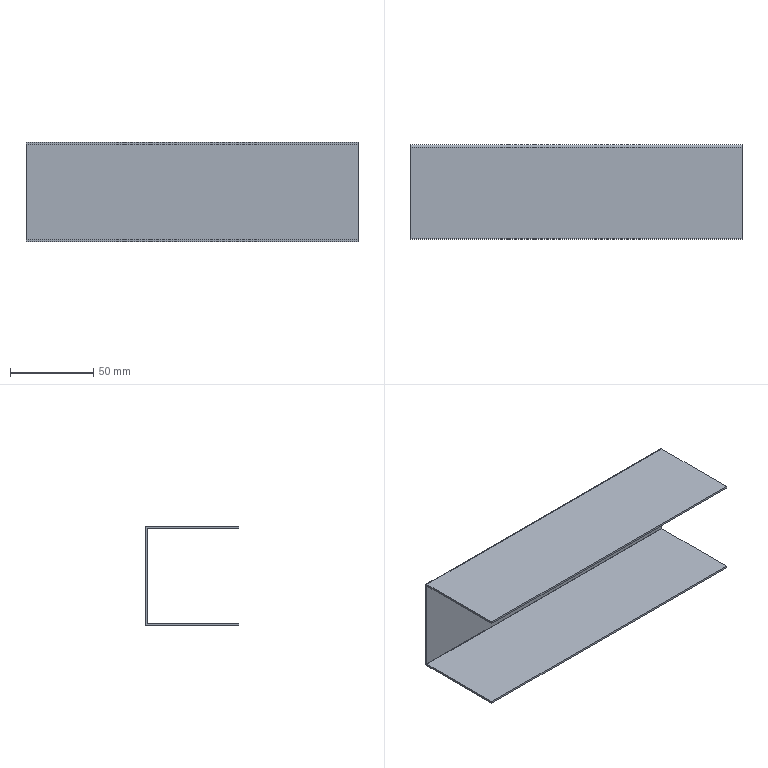Component | SolidWorks | WeldmentDrawing-1_DrawerBoxBracket-1 | 1 solid | 22 faces | box 200 x 56.6 x 60 mm | volume 40848 mm3 | plane 18 | cylinder 4 | commonest cylinder face diameters 2.6 x2 0.2 x2
STEP:
#1=CARTESIAN_POINT('',(-5.191,-11.825,-0.3425));
#2=VERTEX_POINT('',#1);
#3=CARTESIAN_POINT('',(-5.191,-11.825,1.917));
#4=VERTEX_POINT('',#3);
#5=CARTESIAN_POINT('',(-5.191,-11.825,1.969));
#6=DIRECTION('',(0.,0.,1.));
#7=VECTOR('',#6,39.37);
#8=LINE('',#5,#7);
#9=EDGE_CURVE('',#2,#4,#8,.T.);
#10=ORIENTED_EDGE('',*,*,#9,.F.);
#11=CARTESIAN_POINT('',(2.683,-11.825,-0.3425));
#12=VERTEX_POINT('',#11);
#13=CARTESIAN_POINT('',(2.683,-11.825,-0.3425));
#14=DIRECTION('',(-1.,0.,0.));
#15=VECTOR('',#14,39.37);
#16=LINE('',#13,#15);
#17=EDGE_CURVE('',#12,#2,#16,.T.);
#18=ORIENTED_EDGE('',*,*,#17,.F.);
#19=CARTESIAN_POINT('',(2.683,-11.825,1.917));
#20=VERTEX_POINT('',#19);
#21=CARTESIAN_POINT('',(2.683,-11.825,1.969));
#22=DIRECTION('',(0.,0.,-1.));
#23=VECTOR('',#22,39.37);
#24=LINE('',#21,#23);
#25=EDGE_CURVE('',#20,#12,#24,.T.);
#26=ORIENTED_EDGE('',*,*,#25,.F.);
#27=CARTESIAN_POINT('',(-5.191,-11.825,1.917));
#28=DIRECTION('',(1.,0.,0.));
#29=VECTOR('',#28,39.37);
#30=LINE('',#27,#29);
#31=EDGE_CURVE('',#4,#20,#30,.T.);
#32=ORIENTED_EDGE('',*,*,#31,.F.);
#33=EDGE_LOOP('',(#10,#18,#26,#32));
#34=FACE_OUTER_BOUND('',#33,.T.);
#35=CARTESIAN_POINT('',(-2.423,-11.825,0.8285));
#36=DIRECTION('',(0.,-1.,0.));
#37=DIRECTION('',(0.,0.,-1.));
#38=AXIS2_PLACEMENT_3D('',#35,#36,#37);
#39=PLANE('',#38);
#40=ADVANCED_FACE('',(#34),#39,.T.);
#41=CARTESIAN_POINT('',(2.683,-11.778,-0.3425));
#42=VERTEX_POINT('',#41);
#43=CARTESIAN_POINT('',(-5.191,-11.778,-0.3425));
#44=VERTEX_POINT('',#43);
#45=CARTESIAN_POINT('',(2.683,-11.778,-0.3425));
#46=DIRECTION('',(-1.,0.,0.));
#47=VECTOR('',#46,39.37);
#48=LINE('',#45,#47);
#49=EDGE_CURVE('',#42,#44,#48,.T.);
#50=ORIENTED_EDGE('',*,*,#49,.T.);
#51=CARTESIAN_POINT('',(-5.191,-11.778,1.917));
#52=VERTEX_POINT('',#51);
#53=CARTESIAN_POINT('',(-5.191,-11.778,1.969));
#54=DIRECTION('',(0.,0.,1.));
#55=VECTOR('',#54,39.37);
#56=LINE('',#53,#55);
#57=EDGE_CURVE('',#44,#52,#56,.T.);
#58=ORIENTED_EDGE('',*,*,#57,.T.);
#59=CARTESIAN_POINT('',(2.683,-11.778,1.917));
#60=VERTEX_POINT('',#59);
#61=CARTESIAN_POINT('',(-5.191,-11.778,1.917));
#62=DIRECTION('',(1.,0.,0.));
#63=VECTOR('',#62,39.37);
#64=LINE('',#61,#63);
#65=EDGE_CURVE('',#52,#60,#64,.T.);
#66=ORIENTED_EDGE('',*,*,#65,.T.);
#67=CARTESIAN_POINT('',(2.683,-11.778,1.969));
#68=DIRECTION('',(0.,0.,-1.));
#69=VECTOR('',#68,39.37);
#70=LINE('',#67,#69);
#71=EDGE_CURVE('',#60,#42,#70,.T.);
#72=ORIENTED_EDGE('',*,*,#71,.T.);
#73=EDGE_LOOP('',(#50,#58,#66,#72));
#74=FACE_OUTER_BOUND('',#73,.T.);
#75=CARTESIAN_POINT('',(-2.423,-11.778,0.8285));
#76=DIRECTION('',(0.,-1.,0.));
#77=DIRECTION('',(0.,0.,-1.));
#78=AXIS2_PLACEMENT_3D('',#75,#76,#77);
#79=PLANE('',#78);
#80=ADVANCED_FACE('',(#74),#79,.F.);
#81=ORIENTED_EDGE('',*,*,#25,.T.);
#82=CARTESIAN_POINT('',(2.683,-11.825,-0.3425));
#83=DIRECTION('',(0.,1.,0.));
#84=VECTOR('',#83,39.37);
#85=LINE('',#82,#84);
#86=EDGE_CURVE('',#12,#42,#85,.T.);
#87=ORIENTED_EDGE('',*,*,#86,.T.);
#88=ORIENTED_EDGE('',*,*,#71,.F.);
#89=CARTESIAN_POINT('',(2.683,-11.825,1.917));
#90=DIRECTION('',(0.,1.,0.));
#91=VECTOR('',#90,39.37);
#92=LINE('',#89,#91);
#93=EDGE_CURVE('',#20,#60,#92,.T.);
#94=ORIENTED_EDGE('',*,*,#93,.F.);
#95=EDGE_LOOP('',(#81,#87,#88,#94));
#96=FACE_OUTER_BOUND('',#95,.T.);
#97=CARTESIAN_POINT('',(2.683,-11.825,1.969));
#98=DIRECTION('',(1.,0.,0.));
#99=DIRECTION('',(0.,0.,-1.));
#100=AXIS2_PLACEMENT_3D('',#97,#98,#99);
#101=PLANE('',#100);
#102=ADVANCED_FACE('',(#96),#101,.T.);
#103=CARTESIAN_POINT('',(-5.191,-11.825,-0.3425));
#104=DIRECTION('',(0.,1.,0.));
#105=VECTOR('',#104,39.37);
#106=LINE('',#103,#105);
#107=EDGE_CURVE('',#2,#44,#106,.T.);
#108=ORIENTED_EDGE('',*,*,#107,.F.);
#109=ORIENTED_EDGE('',*,*,#9,.T.);
#110=CARTESIAN_POINT('',(-5.191,-11.825,1.917));
#111=DIRECTION('',(0.,1.,0.));
#112=VECTOR('',#111,39.37);
#113=LINE('',#110,#112);
#114=EDGE_CURVE('',#4,#52,#113,.T.);
#115=ORIENTED_EDGE('',*,*,#114,.T.);
#116=ORIENTED_EDGE('',*,*,#57,.F.);
#117=EDGE_LOOP('',(#108,#109,#115,#116));
#118=FACE_OUTER_BOUND('',#117,.T.);
#119=CARTESIAN_POINT('',(-5.191,-11.825,1.969));
#120=DIRECTION('',(-1.,0.,0.));
#121=DIRECTION('',(0.,0.,1.));
#122=AXIS2_PLACEMENT_3D('',#119,#120,#121);
#123=PLANE('',#122);
#124=ADVANCED_FACE('',(#118),#123,.T.);
#125=CARTESIAN_POINT('',(2.683,-11.829,1.921));
#126=VERTEX_POINT('',#125);
#127=CARTESIAN_POINT('',(2.683,-11.829,1.969));
#128=VERTEX_POINT('',#127);
#129=CARTESIAN_POINT('',(2.683,-11.829,1.969));
#130=DIRECTION('',(0.,0.,1.));
#131=VECTOR('',#130,39.37);
#132=LINE('',#129,#131);
#133=EDGE_CURVE('',#126,#128,#132,.T.);
#134=ORIENTED_EDGE('',*,*,#133,.F.);
#135=CARTESIAN_POINT('',(2.683,-11.829,1.917));
#136=DIRECTION('',(1.,0.,0.));
#137=DIRECTION('',(0.,0.,1.));
#138=AXIS2_PLACEMENT_3D('',#135,#136,#137);
#139=CIRCLE('',#138,0.003937);
#140=EDGE_CURVE('',#20,#126,#139,.T.);
#141=ORIENTED_EDGE('',*,*,#140,.F.);
#142=ORIENTED_EDGE('',*,*,#93,.T.);
#143=CARTESIAN_POINT('',(2.683,-11.829,1.917));
#144=DIRECTION('',(1.,0.,0.));
#145=DIRECTION('',(0.,-0.,1.));
#146=AXIS2_PLACEMENT_3D('',#143,#144,#145);
#147=CIRCLE('',#146,0.05118);
#148=EDGE_CURVE('',#60,#128,#147,.T.);
#149=ORIENTED_EDGE('',*,*,#148,.T.);
#150=EDGE_LOOP('',(#134,#141,#142,#149));
#151=FACE_OUTER_BOUND('',#150,.T.);
#152=CARTESIAN_POINT('',(2.683,-11.829,1.917));
#153=DIRECTION('',(1.,0.,0.));
#154=DIRECTION('',(0.,0.,-1.));
#155=AXIS2_PLACEMENT_3D('',#152,#153,#154);
#156=PLANE('',#155);
#157=ADVANCED_FACE('',(#151),#156,.T.);
#158=CARTESIAN_POINT('',(-5.191,-11.829,1.921));
#159=VERTEX_POINT('',#158);
#160=CARTESIAN_POINT('',(-5.191,-11.829,1.917));
#161=DIRECTION('',(-1.,0.,0.));
#162=DIRECTION('',(0.,0.,1.));
#163=AXIS2_PLACEMENT_3D('',#160,#161,#162);
#164=CIRCLE('',#163,0.003937);
#165=EDGE_CURVE('',#159,#4,#164,.T.);
#166=ORIENTED_EDGE('',*,*,#165,.F.);
#167=CARTESIAN_POINT('',(-5.191,-11.829,1.969));
#168=VERTEX_POINT('',#167);
#169=CARTESIAN_POINT('',(-5.191,-11.829,1.921));
#170=DIRECTION('',(0.,0.,1.));
#171=VECTOR('',#170,39.37);
#172=LINE('',#169,#171);
#173=EDGE_CURVE('',#159,#168,#172,.T.);
#174=ORIENTED_EDGE('',*,*,#173,.T.);
#175=CARTESIAN_POINT('',(-5.191,-11.829,1.917));
#176=DIRECTION('',(-1.,0.,0.));
#177=DIRECTION('',(0.,0.,1.));
#178=AXIS2_PLACEMENT_3D('',#175,#176,#177);
#179=CIRCLE('',#178,0.05118);
#180=EDGE_CURVE('',#168,#52,#179,.T.);
#181=ORIENTED_EDGE('',*,*,#180,.T.);
#182=ORIENTED_EDGE('',*,*,#114,.F.);
#183=EDGE_LOOP('',(#166,#174,#181,#182));
#184=FACE_OUTER_BOUND('',#183,.T.);
#185=CARTESIAN_POINT('',(-5.191,-11.829,1.917));
#186=DIRECTION('',(1.,0.,0.));
#187=DIRECTION('',(0.,0.,-1.));
#188=AXIS2_PLACEMENT_3D('',#185,#186,#187);
#189=PLANE('',#188);
#190=ADVANCED_FACE('',(#184),#189,.F.);
#191=ORIENTED_EDGE('',*,*,#65,.F.);
#192=ORIENTED_EDGE('',*,*,#180,.F.);
#193=CARTESIAN_POINT('',(-2.423,-11.829,1.969));
#194=DIRECTION('',(-1.,0.,0.));
#195=VECTOR('',#194,39.37);
#196=LINE('',#193,#195);
#197=EDGE_CURVE('',#128,#168,#196,.T.);
#198=ORIENTED_EDGE('',*,*,#197,.F.);
#199=ORIENTED_EDGE('',*,*,#148,.F.);
#200=EDGE_LOOP('',(#191,#192,#198,#199));
#201=FACE_OUTER_BOUND('',#200,.T.);
#202=CARTESIAN_POINT('',(-5.191,-11.829,1.917));
#203=DIRECTION('',(-1.,0.,0.));
#204=DIRECTION('',(0.,0.,1.));
#205=AXIS2_PLACEMENT_3D('',#202,#203,#204);
#206=CYLINDRICAL_SURFACE('',#205,0.05118);
#207=ADVANCED_FACE('',(#201),#206,.T.);
#208=ORIENTED_EDGE('',*,*,#31,.T.);
#209=ORIENTED_EDGE('',*,*,#140,.T.);
#210=CARTESIAN_POINT('',(2.683,-11.829,1.921));
#211=DIRECTION('',(-1.,0.,0.));
#212=VECTOR('',#211,39.37);
#213=LINE('',#210,#212);
#214=EDGE_CURVE('',#126,#159,#213,.T.);
#215=ORIENTED_EDGE('',*,*,#214,.T.);
#216=ORIENTED_EDGE('',*,*,#165,.T.);
#217=EDGE_LOOP('',(#208,#209,#215,#216));
#218=FACE_OUTER_BOUND('',#217,.T.);
#219=CARTESIAN_POINT('',(-5.191,-11.829,1.917));
#220=DIRECTION('',(-1.,0.,0.));
#221=DIRECTION('',(0.,0.,1.));
#222=AXIS2_PLACEMENT_3D('',#219,#220,#221);
#223=CYLINDRICAL_SURFACE('',#222,0.003937);
#224=ADVANCED_FACE('',(#218),#223,.F.);
#225=CARTESIAN_POINT('',(-5.191,-14.006,1.969));
#226=VERTEX_POINT('',#225);
#227=CARTESIAN_POINT('',(-5.191,-11.825,1.969));
#228=DIRECTION('',(0.,1.,-0.));
#229=VECTOR('',#228,39.37);
#230=LINE('',#227,#229);
#231=EDGE_CURVE('',#226,#168,#230,.T.);
#232=ORIENTED_EDGE('',*,*,#231,.T.);
#233=ORIENTED_EDGE('',*,*,#173,.F.);
#234=CARTESIAN_POINT('',(-5.191,-14.006,1.921));
#235=VERTEX_POINT('',#234);
#236=CARTESIAN_POINT('',(-5.191,-11.778,1.921));
#237=DIRECTION('',(0.,1.,-0.));
#238=VECTOR('',#237,39.37);
#239=LINE('',#236,#238);
#240=EDGE_CURVE('',#235,#159,#239,.T.);
#241=ORIENTED_EDGE('',*,*,#240,.F.);
#242=CARTESIAN_POINT('',(-5.191,-14.006,1.969));
#243=DIRECTION('',(0.,-0.,-1.));
#244=VECTOR('',#243,39.37);
#245=LINE('',#242,#244);
#246=EDGE_CURVE('',#226,#235,#245,.T.);
#247=ORIENTED_EDGE('',*,*,#246,.F.);
#248=EDGE_LOOP('',(#232,#233,#241,#247));
#249=FACE_OUTER_BOUND('',#248,.T.);
#250=CARTESIAN_POINT('',(-5.191,-11.825,1.969));
#251=DIRECTION('',(-1.,0.,0.));
#252=DIRECTION('',(0.,0.,1.));
#253=AXIS2_PLACEMENT_3D('',#250,#251,#252);
#254=PLANE('',#253);
#255=ADVANCED_FACE('',(#249),#254,.T.);
#256=CARTESIAN_POINT('',(2.683,-14.006,1.921));
#257=VERTEX_POINT('',#256);
#258=CARTESIAN_POINT('',(2.683,-11.778,1.921));
#259=DIRECTION('',(0.,-1.,0.));
#260=VECTOR('',#259,39.37);
#261=LINE('',#258,#260);
#262=EDGE_CURVE('',#126,#257,#261,.T.);
#263=ORIENTED_EDGE('',*,*,#262,.F.);
#264=ORIENTED_EDGE('',*,*,#133,.T.);
#265=CARTESIAN_POINT('',(2.683,-14.006,1.969));
#266=VERTEX_POINT('',#265);
#267=CARTESIAN_POINT('',(2.683,-14.006,1.969));
#268=DIRECTION('',(0.,-1.,0.));
#269=VECTOR('',#268,39.37);
#270=LINE('',#267,#269);
#271=EDGE_CURVE('',#128,#266,#270,.T.);
#272=ORIENTED_EDGE('',*,*,#271,.T.);
#273=CARTESIAN_POINT('',(2.683,-14.006,1.969));
#274=DIRECTION('',(0.,-0.,-1.));
#275=VECTOR('',#274,39.37);
#276=LINE('',#273,#275);
#277=EDGE_CURVE('',#266,#257,#276,.T.);
#278=ORIENTED_EDGE('',*,*,#277,.T.);
#279=EDGE_LOOP('',(#263,#264,#272,#278));
#280=FACE_OUTER_BOUND('',#279,.T.);
#281=CARTESIAN_POINT('',(2.683,-14.006,1.969));
#282=DIRECTION('',(1.,0.,0.));
#283=DIRECTION('',(0.,0.,-1.));
#284=AXIS2_PLACEMENT_3D('',#281,#282,#283);
#285=PLANE('',#284);
#286=ADVANCED_FACE('',(#280),#285,.T.);
#287=ORIENTED_EDGE('',*,*,#271,.F.);
#288=ORIENTED_EDGE('',*,*,#197,.T.);
#289=ORIENTED_EDGE('',*,*,#231,.F.);
#290=CARTESIAN_POINT('',(-5.191,-14.006,1.969));
#291=DIRECTION('',(-1.,0.,0.));
#292=VECTOR('',#291,39.37);
#293=LINE('',#290,#292);
#294=EDGE_CURVE('',#266,#226,#293,.T.);
#295=ORIENTED_EDGE('',*,*,#294,.F.);
#296=EDGE_LOOP('',(#287,#288,#289,#295));
#297=FACE_OUTER_BOUND('',#296,.T.);
#298=CARTESIAN_POINT('',(-2.423,-11.778,1.969));
#299=DIRECTION('',(0.,0.,1.));
#300=DIRECTION('',(0.,-1.,0.));
#301=AXIS2_PLACEMENT_3D('',#298,#299,#300);
#302=PLANE('',#301);
#303=ADVANCED_FACE('',(#297),#302,.T.);
#304=ORIENTED_EDGE('',*,*,#214,.F.);
#305=ORIENTED_EDGE('',*,*,#262,.T.);
#306=CARTESIAN_POINT('',(-2.423,-14.006,1.921));
#307=DIRECTION('',(-1.,0.,0.));
#308=VECTOR('',#307,39.37);
#309=LINE('',#306,#308);
#310=EDGE_CURVE('',#257,#235,#309,.T.);
#311=ORIENTED_EDGE('',*,*,#310,.T.);
#312=ORIENTED_EDGE('',*,*,#240,.T.);
#313=EDGE_LOOP('',(#304,#305,#311,#312));
#314=FACE_OUTER_BOUND('',#313,.T.);
#315=CARTESIAN_POINT('',(-2.423,-11.778,1.921));
#316=DIRECTION('',(0.,0.,1.));
#317=DIRECTION('',(0.,-1.,0.));
#318=AXIS2_PLACEMENT_3D('',#315,#316,#317);
#319=PLANE('',#318);
#320=ADVANCED_FACE('',(#314),#319,.F.);
#321=ORIENTED_EDGE('',*,*,#310,.F.);
#322=ORIENTED_EDGE('',*,*,#277,.F.);
#323=ORIENTED_EDGE('',*,*,#294,.T.);
#324=ORIENTED_EDGE('',*,*,#246,.T.);
#325=EDGE_LOOP('',(#321,#322,#323,#324));
#326=FACE_OUTER_BOUND('',#325,.T.);
#327=CARTESIAN_POINT('',(-5.191,-14.006,1.969));
#328=DIRECTION('',(0.,-1.,0.));
#329=DIRECTION('',(0.,-0.,-1.));
#330=AXIS2_PLACEMENT_3D('',#327,#328,#329);
#331=PLANE('',#330);
#332=ADVANCED_FACE('',(#326),#331,.T.);
#333=CARTESIAN_POINT('',(-5.191,-11.829,-0.3464));
#334=VERTEX_POINT('',#333);
#335=CARTESIAN_POINT('',(-5.191,-11.829,-0.3937));
#336=VERTEX_POINT('',#335);
#337=CARTESIAN_POINT('',(-5.191,-11.829,-0.3937));
#338=DIRECTION('',(0.,0.,-1.));
#339=VECTOR('',#338,39.37);
#340=LINE('',#337,#339);
#341=EDGE_CURVE('',#334,#336,#340,.T.);
#342=ORIENTED_EDGE('',*,*,#341,.F.);
#343=CARTESIAN_POINT('',(-5.191,-11.829,-0.3425));
#344=DIRECTION('',(-1.,0.,0.));
#345=DIRECTION('',(0.,0.,-1.));
#346=AXIS2_PLACEMENT_3D('',#343,#344,#345);
#347=CIRCLE('',#346,0.003937);
#348=EDGE_CURVE('',#2,#334,#347,.T.);
#349=ORIENTED_EDGE('',*,*,#348,.F.);
#350=ORIENTED_EDGE('',*,*,#107,.T.);
#351=CARTESIAN_POINT('',(-5.191,-11.829,-0.3425));
#352=DIRECTION('',(-1.,0.,0.));
#353=DIRECTION('',(0.,0.,-1.));
#354=AXIS2_PLACEMENT_3D('',#351,#352,#353);
#355=CIRCLE('',#354,0.05118);
#356=EDGE_CURVE('',#44,#336,#355,.T.);
#357=ORIENTED_EDGE('',*,*,#356,.T.);
#358=EDGE_LOOP('',(#342,#349,#350,#357));
#359=FACE_OUTER_BOUND('',#358,.T.);
#360=CARTESIAN_POINT('',(-5.191,-11.829,-0.3425));
#361=DIRECTION('',(-1.,0.,0.));
#362=DIRECTION('',(0.,0.,1.));
#363=AXIS2_PLACEMENT_3D('',#360,#361,#362);
#364=PLANE('',#363);
#365=ADVANCED_FACE('',(#359),#364,.T.);
#366=CARTESIAN_POINT('',(2.683,-11.829,-0.3464));
#367=VERTEX_POINT('',#366);
#368=CARTESIAN_POINT('',(2.683,-11.829,-0.3425));
#369=DIRECTION('',(1.,0.,0.));
#370=DIRECTION('',(0.,0.,-1.));
#371=AXIS2_PLACEMENT_3D('',#368,#369,#370);
#372=CIRCLE('',#371,0.003937);
#373=EDGE_CURVE('',#367,#12,#372,.T.);
#374=ORIENTED_EDGE('',*,*,#373,.F.);
#375=CARTESIAN_POINT('',(2.683,-11.829,-0.3937));
#376=VERTEX_POINT('',#375);
#377=CARTESIAN_POINT('',(2.683,-11.829,-0.3464));
#378=DIRECTION('',(0.,0.,-1.));
#379=VECTOR('',#378,39.37);
#380=LINE('',#377,#379);
#381=EDGE_CURVE('',#367,#376,#380,.T.);
#382=ORIENTED_EDGE('',*,*,#381,.T.);
#383=CARTESIAN_POINT('',(2.683,-11.829,-0.3425));
#384=DIRECTION('',(1.,0.,0.));
#385=DIRECTION('',(0.,0.,-1.));
#386=AXIS2_PLACEMENT_3D('',#383,#384,#385);
#387=CIRCLE('',#386,0.05118);
#388=EDGE_CURVE('',#376,#42,#387,.T.);
#389=ORIENTED_EDGE('',*,*,#388,.T.);
#390=ORIENTED_EDGE('',*,*,#86,.F.);
#391=EDGE_LOOP('',(#374,#382,#389,#390));
#392=FACE_OUTER_BOUND('',#391,.T.);
#393=CARTESIAN_POINT('',(2.683,-11.829,-0.3425));
#394=DIRECTION('',(-1.,0.,0.));
#395=DIRECTION('',(0.,0.,1.));
#396=AXIS2_PLACEMENT_3D('',#393,#394,#395);
#397=PLANE('',#396);
#398=ADVANCED_FACE('',(#392),#397,.F.);
#399=ORIENTED_EDGE('',*,*,#49,.F.);
#400=ORIENTED_EDGE('',*,*,#388,.F.);
#401=CARTESIAN_POINT('',(-5.191,-11.829,-0.3937));
#402=DIRECTION('',(-1.,0.,0.));
#403=VECTOR('',#402,39.37);
#404=LINE('',#401,#403);
#405=EDGE_CURVE('',#376,#336,#404,.T.);
#406=ORIENTED_EDGE('',*,*,#405,.T.);
#407=ORIENTED_EDGE('',*,*,#356,.F.);
#408=EDGE_LOOP('',(#399,#400,#406,#407));
#409=FACE_OUTER_BOUND('',#408,.T.);
#410=CARTESIAN_POINT('',(2.683,-11.829,-0.3425));
#411=DIRECTION('',(1.,0.,0.));
#412=DIRECTION('',(0.,0.,-1.));
#413=AXIS2_PLACEMENT_3D('',#410,#411,#412);
#414=CYLINDRICAL_SURFACE('',#413,0.05118);
#415=ADVANCED_FACE('',(#409),#414,.T.);
#416=ORIENTED_EDGE('',*,*,#17,.T.);
#417=ORIENTED_EDGE('',*,*,#348,.T.);
#418=CARTESIAN_POINT('',(-5.191,-11.829,-0.3464));
#419=DIRECTION('',(1.,-0.,-0.));
#420=VECTOR('',#419,39.37);
#421=LINE('',#418,#420);
#422=EDGE_CURVE('',#334,#367,#421,.T.);
#423=ORIENTED_EDGE('',*,*,#422,.T.);
#424=ORIENTED_EDGE('',*,*,#373,.T.);
#425=EDGE_LOOP('',(#416,#417,#423,#424));
#426=FACE_OUTER_BOUND('',#425,.T.);
#427=CARTESIAN_POINT('',(2.683,-11.829,-0.3425));
#428=DIRECTION('',(1.,0.,0.));
#429=DIRECTION('',(0.,0.,-1.));
#430=AXIS2_PLACEMENT_3D('',#427,#428,#429);
#431=CYLINDRICAL_SURFACE('',#430,0.003937);
#432=ADVANCED_FACE('',(#426),#431,.F.);
#433=CARTESIAN_POINT('',(-5.191,-14.006,-0.3464));
#434=VERTEX_POINT('',#433);
#435=CARTESIAN_POINT('',(-5.191,-11.778,-0.3464));
#436=DIRECTION('',(0.,-1.,-0.));
#437=VECTOR('',#436,39.37);
#438=LINE('',#435,#437);
#439=EDGE_CURVE('',#334,#434,#438,.T.);
#440=ORIENTED_EDGE('',*,*,#439,.F.);
#441=ORIENTED_EDGE('',*,*,#341,.T.);
#442=CARTESIAN_POINT('',(-5.191,-14.006,-0.3937));
#443=VERTEX_POINT('',#442);
#444=CARTESIAN_POINT('',(-5.191,-11.825,-0.3937));
#445=DIRECTION('',(0.,-1.,-0.));
#446=VECTOR('',#445,39.37);
#447=LINE('',#444,#446);
#448=EDGE_CURVE('',#336,#443,#447,.T.);
#449=ORIENTED_EDGE('',*,*,#448,.T.);
#450=CARTESIAN_POINT('',(-5.191,-14.006,-0.3937));
#451=DIRECTION('',(0.,-0.,1.));
#452=VECTOR('',#451,39.37);
#453=LINE('',#450,#452);
#454=EDGE_CURVE('',#443,#434,#453,.T.);
#455=ORIENTED_EDGE('',*,*,#454,.T.);
#456=EDGE_LOOP('',(#440,#441,#449,#455));
#457=FACE_OUTER_BOUND('',#456,.T.);
#458=CARTESIAN_POINT('',(-5.191,-11.825,-0.3937));
#459=DIRECTION('',(-1.,0.,0.));
#460=DIRECTION('',(0.,0.,1.));
#461=AXIS2_PLACEMENT_3D('',#458,#459,#460);
#462=PLANE('',#461);
#463=ADVANCED_FACE('',(#457),#462,.T.);
#464=CARTESIAN_POINT('',(2.683,-14.006,-0.3937));
#465=VERTEX_POINT('',#464);
#466=CARTESIAN_POINT('',(2.683,-14.006,-0.3937));
#467=DIRECTION('',(0.,1.,0.));
#468=VECTOR('',#467,39.37);
#469=LINE('',#466,#468);
#470=EDGE_CURVE('',#465,#376,#469,.T.);
#471=ORIENTED_EDGE('',*,*,#470,.T.);
#472=ORIENTED_EDGE('',*,*,#381,.F.);
#473=CARTESIAN_POINT('',(2.683,-14.006,-0.3464));
#474=VERTEX_POINT('',#473);
#475=CARTESIAN_POINT('',(2.683,-11.778,-0.3464));
#476=DIRECTION('',(0.,1.,0.));
#477=VECTOR('',#476,39.37);
#478=LINE('',#475,#477);
#479=EDGE_CURVE('',#474,#367,#478,.T.);
#480=ORIENTED_EDGE('',*,*,#479,.F.);
#481=CARTESIAN_POINT('',(2.683,-14.006,-0.3937));
#482=DIRECTION('',(0.,-0.,1.));
#483=VECTOR('',#482,39.37);
#484=LINE('',#481,#483);
#485=EDGE_CURVE('',#465,#474,#484,.T.);
#486=ORIENTED_EDGE('',*,*,#485,.F.);
#487=EDGE_LOOP('',(#471,#472,#480,#486));
#488=FACE_OUTER_BOUND('',#487,.T.);
#489=CARTESIAN_POINT('',(2.683,-14.006,-0.3937));
#490=DIRECTION('',(1.,0.,0.));
#491=DIRECTION('',(0.,0.,-1.));
#492=AXIS2_PLACEMENT_3D('',#489,#490,#491);
#493=PLANE('',#492);
#494=ADVANCED_FACE('',(#488),#493,.T.);
#495=ORIENTED_EDGE('',*,*,#405,.F.);
#496=ORIENTED_EDGE('',*,*,#470,.F.);
#497=CARTESIAN_POINT('',(-5.191,-14.006,-0.3937));
#498=DIRECTION('',(1.,0.,0.));
#499=VECTOR('',#498,39.37);
#500=LINE('',#497,#499);
#501=EDGE_CURVE('',#443,#465,#500,.T.);
#502=ORIENTED_EDGE('',*,*,#501,.F.);
#503=ORIENTED_EDGE('',*,*,#448,.F.);
#504=EDGE_LOOP('',(#495,#496,#502,#503));
#505=FACE_OUTER_BOUND('',#504,.T.);
#506=CARTESIAN_POINT('',(-2.423,-11.778,-0.3937));
#507=DIRECTION('',(0.,-0.,1.));
#508=DIRECTION('',(0.,-1.,-0.));
#509=AXIS2_PLACEMENT_3D('',#506,#507,#508);
#510=PLANE('',#509);
#511=ADVANCED_FACE('',(#505),#510,.F.);
#512=ORIENTED_EDGE('',*,*,#479,.T.);
#513=ORIENTED_EDGE('',*,*,#422,.F.);
#514=ORIENTED_EDGE('',*,*,#439,.T.);
#515=CARTESIAN_POINT('',(-2.423,-14.006,-0.3464));
#516=DIRECTION('',(1.,0.,0.));
#517=VECTOR('',#516,39.37);
#518=LINE('',#515,#517);
#519=EDGE_CURVE('',#434,#474,#518,.T.);
#520=ORIENTED_EDGE('',*,*,#519,.T.);
#521=EDGE_LOOP('',(#512,#513,#514,#520));
#522=FACE_OUTER_BOUND('',#521,.T.);
#523=CARTESIAN_POINT('',(-2.423,-11.778,-0.3464));
#524=DIRECTION('',(0.,-0.,1.));
#525=DIRECTION('',(0.,-1.,-0.));
#526=AXIS2_PLACEMENT_3D('',#523,#524,#525);
#527=PLANE('',#526);
#528=ADVANCED_FACE('',(#522),#527,.T.);
#529=ORIENTED_EDGE('',*,*,#519,.F.);
#530=ORIENTED_EDGE('',*,*,#454,.F.);
#531=ORIENTED_EDGE('',*,*,#501,.T.);
#532=ORIENTED_EDGE('',*,*,#485,.T.);
#533=EDGE_LOOP('',(#529,#530,#531,#532));
#534=FACE_OUTER_BOUND('',#533,.T.);
#535=CARTESIAN_POINT('',(-5.191,-14.006,-0.3937));
#536=DIRECTION('',(0.,-1.,-0.));
#537=DIRECTION('',(0.,0.,-1.));
#538=AXIS2_PLACEMENT_3D('',#535,#536,#537);
#539=PLANE('',#538);
#540=ADVANCED_FACE('',(#534),#539,.T.);
#541=CLOSED_SHELL('',(#40,#80,#102,#124,#157,#190,#207,#224,#255,#286,#303,#320,#332,#365,#398,#415,#432,#463,#494,#511,#528,#540));
#542=MANIFOLD_SOLID_BREP('',#541);
#543=CARTESIAN_POINT('',(0.,0.,0.));
#544=DIRECTION('',(0.,0.,1.));
#545=DIRECTION('',(1.,0.,0.));
#546=AXIS2_PLACEMENT_3D('',#543,#544,#545);
#547=(LENGTH_UNIT()NAMED_UNIT(*)SI_UNIT($,.METRE.));
#548=LENGTH_MEASURE_WITH_UNIT(LENGTH_MEASURE(0.0254),#547);
#549=DIMENSIONAL_EXPONENTS(1.,0.,0.,0.,0.,0.,0.);
#550=(CONVERSION_BASED_UNIT('',#548)LENGTH_UNIT()NAMED_UNIT(#549));
#551=UNCERTAINTY_MEASURE_WITH_UNIT(LENGTH_MEASURE(0.00001),#550,'','');
#552=(NAMED_UNIT(*)PLANE_ANGLE_UNIT()SI_UNIT($,.RADIAN.));
#553=(NAMED_UNIT(*)SI_UNIT($,.STERADIAN.)SOLID_ANGLE_UNIT());
#554=(GEOMETRIC_REPRESENTATION_CONTEXT(3)GLOBAL_UNCERTAINTY_ASSIGNED_CONTEXT((#551))GLOBAL_UNIT_ASSIGNED_CONTEXT((#550,#552,#553))REPRESENTATION_CONTEXT('',''));
#555=ADVANCED_BREP_SHAPE_REPRESENTATION('',(#542,#546),#554);
#556=COLOUR_RGB('',0.7922,0.8196,0.9333);
#557=FILL_AREA_STYLE_COLOUR('',#556);
#558=FILL_AREA_STYLE('',(#557));
#559=SURFACE_STYLE_FILL_AREA(#558);
#560=SURFACE_SIDE_STYLE('',(#559));
#561=SURFACE_STYLE_USAGE(.BOTH.,#560);
#562=PRESENTATION_STYLE_ASSIGNMENT((#561));
#563=STYLED_ITEM('',(#562),#542);
#564=(LENGTH_UNIT()NAMED_UNIT(*)SI_UNIT($,.METRE.));
#565=LENGTH_MEASURE_WITH_UNIT(LENGTH_MEASURE(0.0254),#564);
#566=DIMENSIONAL_EXPONENTS(1.,0.,0.,0.,0.,0.,0.);
#567=(CONVERSION_BASED_UNIT('',#565)LENGTH_UNIT()NAMED_UNIT(#566));
#568=UNCERTAINTY_MEASURE_WITH_UNIT(LENGTH_MEASURE(0.00001),#567,'','');
#569=(NAMED_UNIT(*)PLANE_ANGLE_UNIT()SI_UNIT($,.RADIAN.));
#570=(NAMED_UNIT(*)SI_UNIT($,.STERADIAN.)SOLID_ANGLE_UNIT());
#571=(GEOMETRIC_REPRESENTATION_CONTEXT(3)GLOBAL_UNCERTAINTY_ASSIGNED_CONTEXT((#568))GLOBAL_UNIT_ASSIGNED_CONTEXT((#567,#569,#570))REPRESENTATION_CONTEXT('',''));
#572=MECHANICAL_DESIGN_GEOMETRIC_PRESENTATION_REPRESENTATION('',(#563),#571);
#573=PRESENTATION_LAYER_ASSIGNMENT('','',(#563));